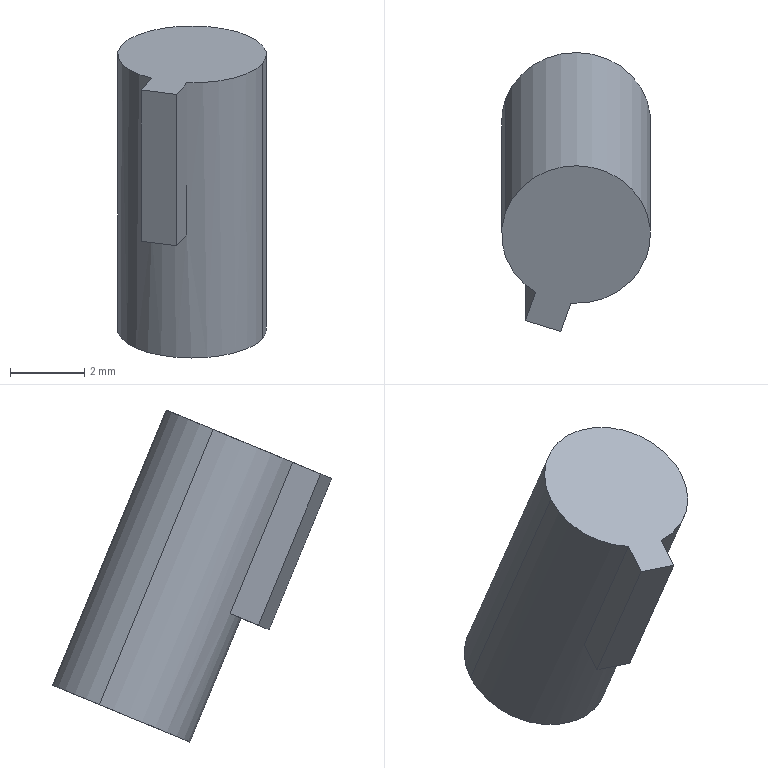Component | SolidWorks | Mirrorpin-2 | 1 solid | 8 faces | box 4 x 7.5 x 8.92 mm | volume 104 mm3 | plane 6 | cylinder 2 | commonest cylinder face diameters 4 x2
STEP:
#1=COLOUR_RGB('',0.7922,0.8196,0.9333);
#2=FILL_AREA_STYLE_COLOUR('',#1);
#3=FILL_AREA_STYLE('',(#2));
#4=SURFACE_STYLE_FILL_AREA(#3);
#5=SURFACE_SIDE_STYLE('',(#4));
#6=SURFACE_STYLE_USAGE(.BOTH.,#5);
#7=PRESENTATION_STYLE_ASSIGNMENT((#6));
#8=CARTESIAN_POINT('',(12.548,-0.9197,2.462));
#9=VERTEX_POINT('',#8);
#10=CARTESIAN_POINT('',(12.698,-0.9657,2.443));
#11=VERTEX_POINT('',#10);
#12=CARTESIAN_POINT('',(12.623,-0.9427,2.452));
#13=DIRECTION('',(0.,0.3818,-0.9242));
#14=DIRECTION('',(0.9487,-0.2921,-0.1207));
#15=AXIS2_PLACEMENT_3D('',#12,#13,#14);
#16=CIRCLE('',#15,0.07874);
#17=EDGE_CURVE('',#9,#11,#16,.T.);
#18=ORIENTED_EDGE('',*,*,#17,.T.);
#19=CARTESIAN_POINT('',(12.698,-0.8455,2.152));
#20=VERTEX_POINT('',#19);
#21=CARTESIAN_POINT('',(12.698,-0.9657,2.443));
#22=DIRECTION('',(0.,0.3818,-0.9242));
#23=VECTOR('',#22,39.37);
#24=LINE('',#21,#23);
#25=EDGE_CURVE('',#11,#20,#24,.T.);
#26=ORIENTED_EDGE('',*,*,#25,.T.);
#27=CARTESIAN_POINT('',(12.548,-0.7995,2.171));
#28=VERTEX_POINT('',#27);
#29=CARTESIAN_POINT('',(12.623,-0.8225,2.161));
#30=DIRECTION('',(0.,0.3818,-0.9242));
#31=DIRECTION('',(0.9487,-0.2921,-0.1207));
#32=AXIS2_PLACEMENT_3D('',#29,#30,#31);
#33=CIRCLE('',#32,0.07874);
#34=EDGE_CURVE('',#28,#20,#33,.T.);
#35=ORIENTED_EDGE('',*,*,#34,.F.);
#36=CARTESIAN_POINT('',(12.548,-0.9197,2.462));
#37=DIRECTION('',(0.,0.3818,-0.9242));
#38=VECTOR('',#37,39.37);
#39=LINE('',#36,#38);
#40=EDGE_CURVE('',#9,#28,#39,.T.);
#41=ORIENTED_EDGE('',*,*,#40,.F.);
#42=EDGE_LOOP('',(#18,#26,#35,#41));
#43=FACE_OUTER_BOUND('',#42,.T.);
#44=CARTESIAN_POINT('',(12.623,-0.9427,2.452));
#45=DIRECTION('',(0.,0.3818,-0.9242));
#46=DIRECTION('',(-0.9487,0.2921,0.1207));
#47=AXIS2_PLACEMENT_3D('',#44,#45,#46);
#48=CYLINDRICAL_SURFACE('',#47,0.07874);
#49=ADVANCED_FACE('',(#43),#48,.T.);
#50=ORIENTED_EDGE('',*,*,#25,.F.);
#51=CARTESIAN_POINT('',(12.617,-1.015,2.422));
#52=VERTEX_POINT('',#51);
#53=CARTESIAN_POINT('',(12.623,-0.9427,2.452));
#54=DIRECTION('',(0.,0.3818,-0.9242));
#55=DIRECTION('',(0.9487,-0.2921,-0.1207));
#56=AXIS2_PLACEMENT_3D('',#53,#54,#55);
#57=CIRCLE('',#56,0.07874);
#58=EDGE_CURVE('',#11,#52,#57,.T.);
#59=ORIENTED_EDGE('',*,*,#58,.T.);
#60=CARTESIAN_POINT('',(12.617,-0.9492,2.262));
#61=VERTEX_POINT('',#60);
#62=CARTESIAN_POINT('',(12.617,-1.015,2.422));
#63=DIRECTION('',(-0.,-0.3818,0.9242));
#64=VECTOR('',#63,39.37);
#65=LINE('',#62,#64);
#66=EDGE_CURVE('',#61,#52,#65,.T.);
#67=ORIENTED_EDGE('',*,*,#66,.F.);
#68=CARTESIAN_POINT('',(12.58,-0.9377,2.267));
#69=VERTEX_POINT('',#68);
#70=CARTESIAN_POINT('',(12.623,-0.8766,2.292));
#71=DIRECTION('',(0.,0.3818,-0.9242));
#72=DIRECTION('',(0.9487,-0.2921,-0.1207));
#73=AXIS2_PLACEMENT_3D('',#70,#71,#72);
#74=CIRCLE('',#73,0.07874);
#75=EDGE_CURVE('',#61,#69,#74,.T.);
#76=ORIENTED_EDGE('',*,*,#75,.T.);
#77=CARTESIAN_POINT('',(12.58,-1.004,2.427));
#78=VERTEX_POINT('',#77);
#79=CARTESIAN_POINT('',(12.58,-1.004,2.427));
#80=DIRECTION('',(0.,0.3818,-0.9242));
#81=VECTOR('',#80,39.37);
#82=LINE('',#79,#81);
#83=EDGE_CURVE('',#78,#69,#82,.T.);
#84=ORIENTED_EDGE('',*,*,#83,.F.);
#85=CARTESIAN_POINT('',(12.623,-0.9427,2.452));
#86=DIRECTION('',(0.,0.3818,-0.9242));
#87=DIRECTION('',(0.9487,-0.2921,-0.1207));
#88=AXIS2_PLACEMENT_3D('',#85,#86,#87);
#89=CIRCLE('',#88,0.07874);
#90=EDGE_CURVE('',#78,#9,#89,.T.);
#91=ORIENTED_EDGE('',*,*,#90,.T.);
#92=ORIENTED_EDGE('',*,*,#40,.T.);
#93=CARTESIAN_POINT('',(12.623,-0.8225,2.161));
#94=DIRECTION('',(0.,0.3818,-0.9242));
#95=DIRECTION('',(0.9487,-0.2921,-0.1207));
#96=AXIS2_PLACEMENT_3D('',#93,#94,#95);
#97=CIRCLE('',#96,0.07874);
#98=EDGE_CURVE('',#20,#28,#97,.T.);
#99=ORIENTED_EDGE('',*,*,#98,.F.);
#100=EDGE_LOOP('',(#50,#59,#67,#76,#84,#91,#92,#99));
#101=FACE_OUTER_BOUND('',#100,.T.);
#102=CARTESIAN_POINT('',(12.623,-0.9427,2.452));
#103=DIRECTION('',(0.,0.3818,-0.9242));
#104=DIRECTION('',(-0.9487,0.2921,0.1207));
#105=AXIS2_PLACEMENT_3D('',#102,#103,#104);
#106=CYLINDRICAL_SURFACE('',#105,0.07874);
#107=ADVANCED_FACE('',(#101),#106,.T.);
#108=ORIENTED_EDGE('',*,*,#90,.F.);
#109=CARTESIAN_POINT('',(12.569,-1.034,2.415));
#110=VERTEX_POINT('',#109);
#111=CARTESIAN_POINT('',(12.604,-0.937,2.455));
#112=DIRECTION('',(0.3161,0.8768,0.3623));
#113=VECTOR('',#112,39.37);
#114=LINE('',#111,#113);
#115=EDGE_CURVE('',#110,#78,#114,.T.);
#116=ORIENTED_EDGE('',*,*,#115,.F.);
#117=CARTESIAN_POINT('',(12.607,-1.045,2.41));
#118=VERTEX_POINT('',#117);
#119=CARTESIAN_POINT('',(12.569,-1.034,2.415));
#120=DIRECTION('',(-0.9487,0.2921,0.1207));
#121=VECTOR('',#120,39.37);
#122=LINE('',#119,#121);
#123=EDGE_CURVE('',#118,#110,#122,.T.);
#124=ORIENTED_EDGE('',*,*,#123,.F.);
#125=CARTESIAN_POINT('',(12.642,-0.9485,2.45));
#126=DIRECTION('',(-0.3161,-0.8768,-0.3623));
#127=VECTOR('',#126,39.37);
#128=LINE('',#125,#127);
#129=EDGE_CURVE('',#52,#118,#128,.T.);
#130=ORIENTED_EDGE('',*,*,#129,.F.);
#131=ORIENTED_EDGE('',*,*,#58,.F.);
#132=ORIENTED_EDGE('',*,*,#17,.F.);
#133=EDGE_LOOP('',(#108,#116,#124,#130,#131,#132));
#134=FACE_OUTER_BOUND('',#133,.T.);
#135=CARTESIAN_POINT('',(12.623,-0.9427,2.452));
#136=DIRECTION('',(-0.,-0.3818,0.9242));
#137=DIRECTION('',(0.9487,-0.2921,-0.1207));
#138=AXIS2_PLACEMENT_3D('',#135,#136,#137);
#139=PLANE('',#138);
#140=ADVANCED_FACE('',(#134),#139,.T.);
#141=ORIENTED_EDGE('',*,*,#34,.T.);
#142=ORIENTED_EDGE('',*,*,#98,.T.);
#143=EDGE_LOOP('',(#141,#142));
#144=FACE_OUTER_BOUND('',#143,.T.);
#145=CARTESIAN_POINT('',(12.623,-0.8225,2.161));
#146=DIRECTION('',(-0.,-0.3818,0.9242));
#147=DIRECTION('',(0.9487,-0.2921,-0.1207));
#148=AXIS2_PLACEMENT_3D('',#145,#146,#147);
#149=PLANE('',#148);
#150=ADVANCED_FACE('',(#144),#149,.F.);
#151=ORIENTED_EDGE('',*,*,#83,.T.);
#152=CARTESIAN_POINT('',(12.569,-0.9675,2.255));
#153=VERTEX_POINT('',#152);
#154=CARTESIAN_POINT('',(12.604,-0.8708,2.295));
#155=DIRECTION('',(0.3161,0.8768,0.3623));
#156=VECTOR('',#155,39.37);
#157=LINE('',#154,#156);
#158=EDGE_CURVE('',#153,#69,#157,.T.);
#159=ORIENTED_EDGE('',*,*,#158,.F.);
#160=CARTESIAN_POINT('',(12.569,-0.9675,2.255));
#161=DIRECTION('',(-0.,-0.3818,0.9242));
#162=VECTOR('',#161,39.37);
#163=LINE('',#160,#162);
#164=EDGE_CURVE('',#153,#110,#163,.T.);
#165=ORIENTED_EDGE('',*,*,#164,.T.);
#166=ORIENTED_EDGE('',*,*,#115,.T.);
#167=EDGE_LOOP('',(#151,#159,#165,#166));
#168=FACE_OUTER_BOUND('',#167,.T.);
#169=CARTESIAN_POINT('',(12.604,-0.8708,2.295));
#170=DIRECTION('',(-0.9487,0.2921,0.1207));
#171=DIRECTION('',(0.3161,0.8768,0.3623));
#172=AXIS2_PLACEMENT_3D('',#169,#170,#171);
#173=PLANE('',#172);
#174=ADVANCED_FACE('',(#168),#173,.T.);
#175=ORIENTED_EDGE('',*,*,#66,.T.);
#176=ORIENTED_EDGE('',*,*,#129,.T.);
#177=CARTESIAN_POINT('',(12.607,-0.979,2.25));
#178=VERTEX_POINT('',#177);
#179=CARTESIAN_POINT('',(12.607,-0.979,2.25));
#180=DIRECTION('',(-0.,-0.3818,0.9242));
#181=VECTOR('',#180,39.37);
#182=LINE('',#179,#181);
#183=EDGE_CURVE('',#178,#118,#182,.T.);
#184=ORIENTED_EDGE('',*,*,#183,.F.);
#185=CARTESIAN_POINT('',(12.642,-0.8823,2.29));
#186=DIRECTION('',(-0.3161,-0.8768,-0.3623));
#187=VECTOR('',#186,39.37);
#188=LINE('',#185,#187);
#189=EDGE_CURVE('',#61,#178,#188,.T.);
#190=ORIENTED_EDGE('',*,*,#189,.F.);
#191=EDGE_LOOP('',(#175,#176,#184,#190));
#192=FACE_OUTER_BOUND('',#191,.T.);
#193=CARTESIAN_POINT('',(12.642,-0.8823,2.29));
#194=DIRECTION('',(0.9487,-0.2921,-0.1207));
#195=DIRECTION('',(-0.3161,-0.8768,-0.3623));
#196=AXIS2_PLACEMENT_3D('',#193,#194,#195);
#197=PLANE('',#196);
#198=ADVANCED_FACE('',(#192),#197,.T.);
#199=ORIENTED_EDGE('',*,*,#123,.T.);
#200=ORIENTED_EDGE('',*,*,#164,.F.);
#201=CARTESIAN_POINT('',(12.569,-0.9675,2.255));
#202=DIRECTION('',(-0.9487,0.2921,0.1207));
#203=VECTOR('',#202,39.37);
#204=LINE('',#201,#203);
#205=EDGE_CURVE('',#178,#153,#204,.T.);
#206=ORIENTED_EDGE('',*,*,#205,.F.);
#207=ORIENTED_EDGE('',*,*,#183,.T.);
#208=EDGE_LOOP('',(#199,#200,#206,#207));
#209=FACE_OUTER_BOUND('',#208,.T.);
#210=CARTESIAN_POINT('',(12.569,-0.9675,2.255));
#211=DIRECTION('',(-0.3161,-0.8768,-0.3623));
#212=DIRECTION('',(-0.9487,0.2921,0.1207));
#213=AXIS2_PLACEMENT_3D('',#210,#211,#212);
#214=PLANE('',#213);
#215=ADVANCED_FACE('',(#209),#214,.T.);
#216=ORIENTED_EDGE('',*,*,#189,.T.);
#217=ORIENTED_EDGE('',*,*,#205,.T.);
#218=ORIENTED_EDGE('',*,*,#158,.T.);
#219=ORIENTED_EDGE('',*,*,#75,.F.);
#220=EDGE_LOOP('',(#216,#217,#218,#219));
#221=FACE_OUTER_BOUND('',#220,.T.);
#222=CARTESIAN_POINT('',(12.623,-0.8766,2.292));
#223=DIRECTION('',(-0.,-0.3818,0.9242));
#224=DIRECTION('',(0.9487,-0.2921,-0.1207));
#225=AXIS2_PLACEMENT_3D('',#222,#223,#224);
#226=PLANE('',#225);
#227=ADVANCED_FACE('',(#221),#226,.F.);
#228=CLOSED_SHELL('',(#49,#107,#140,#150,#174,#198,#215,#227));
#229=MANIFOLD_SOLID_BREP('',#228);
#230=STYLED_ITEM('',(#7),#229);
#231=PRESENTATION_LAYER_ASSIGNMENT('','',(#230));
#232=CARTESIAN_POINT('',(0.,0.,0.));
#233=DIRECTION('',(0.,0.,1.));
#234=DIRECTION('',(1.,0.,0.));
#235=AXIS2_PLACEMENT_3D('',#232,#233,#234);
#236=(LENGTH_UNIT()NAMED_UNIT(*)SI_UNIT($,.METRE.));
#237=LENGTH_MEASURE_WITH_UNIT(LENGTH_MEASURE(0.0254),#236);
#238=DIMENSIONAL_EXPONENTS(1.,0.,0.,0.,0.,0.,0.);
#239=(CONVERSION_BASED_UNIT('',#237)LENGTH_UNIT()NAMED_UNIT(#238));
#240=UNCERTAINTY_MEASURE_WITH_UNIT(LENGTH_MEASURE(0.00001),#239,'','');
#241=(NAMED_UNIT(*)PLANE_ANGLE_UNIT()SI_UNIT($,.RADIAN.));
#242=(NAMED_UNIT(*)SI_UNIT($,.STERADIAN.)SOLID_ANGLE_UNIT());
#243=(GEOMETRIC_REPRESENTATION_CONTEXT(3)GLOBAL_UNCERTAINTY_ASSIGNED_CONTEXT((#240))GLOBAL_UNIT_ASSIGNED_CONTEXT((#239,#241,#242))REPRESENTATION_CONTEXT('',''));
#244=ADVANCED_BREP_SHAPE_REPRESENTATION('',(#229,#235),#243);
#245=(LENGTH_UNIT()NAMED_UNIT(*)SI_UNIT($,.METRE.));
#246=LENGTH_MEASURE_WITH_UNIT(LENGTH_MEASURE(0.0254),#245);
#247=DIMENSIONAL_EXPONENTS(1.,0.,0.,0.,0.,0.,0.);
#248=(CONVERSION_BASED_UNIT('',#246)LENGTH_UNIT()NAMED_UNIT(#247));
#249=UNCERTAINTY_MEASURE_WITH_UNIT(LENGTH_MEASURE(0.00001),#248,'','');
#250=(NAMED_UNIT(*)PLANE_ANGLE_UNIT()SI_UNIT($,.RADIAN.));
#251=(NAMED_UNIT(*)SI_UNIT($,.STERADIAN.)SOLID_ANGLE_UNIT());
#252=(GEOMETRIC_REPRESENTATION_CONTEXT(3)GLOBAL_UNCERTAINTY_ASSIGNED_CONTEXT((#249))GLOBAL_UNIT_ASSIGNED_CONTEXT((#248,#250,#251))REPRESENTATION_CONTEXT('',''));
#253=MECHANICAL_DESIGN_GEOMETRIC_PRESENTATION_REPRESENTATION('',(#230),#252);